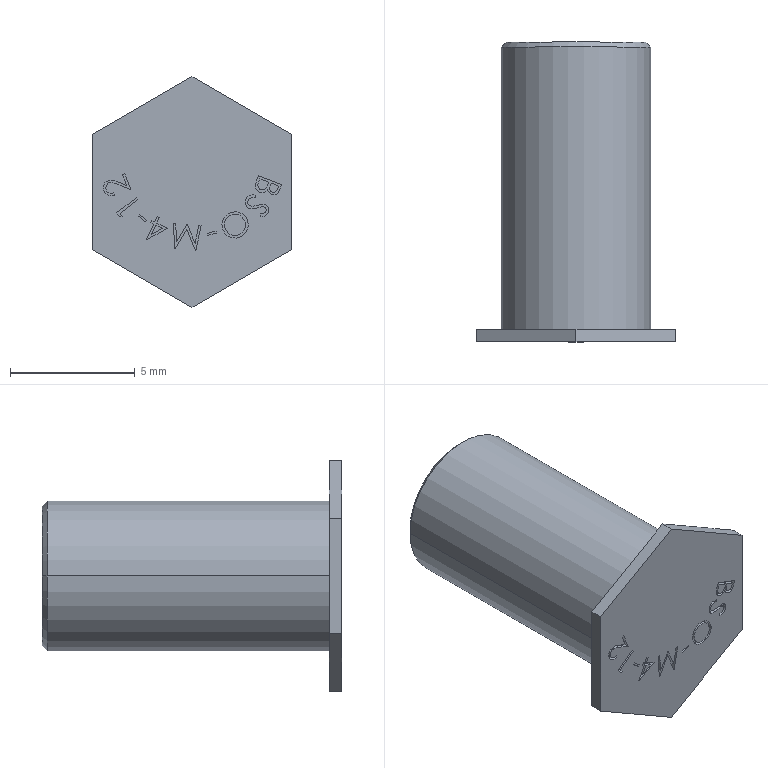Component | SolidWorks | FrontDoorAssembly-1_FrontDoorWelding-1_FrontDoorFrame(Riveted)PG50-02-101-1_BSO-M4-12-10 | 1 solid | 126 faces | volume 207 mm3 | plane 80 | spline 38 | cone 4 | cylinder 4 | commonest cylinder face diameters 4 x2 6 x2